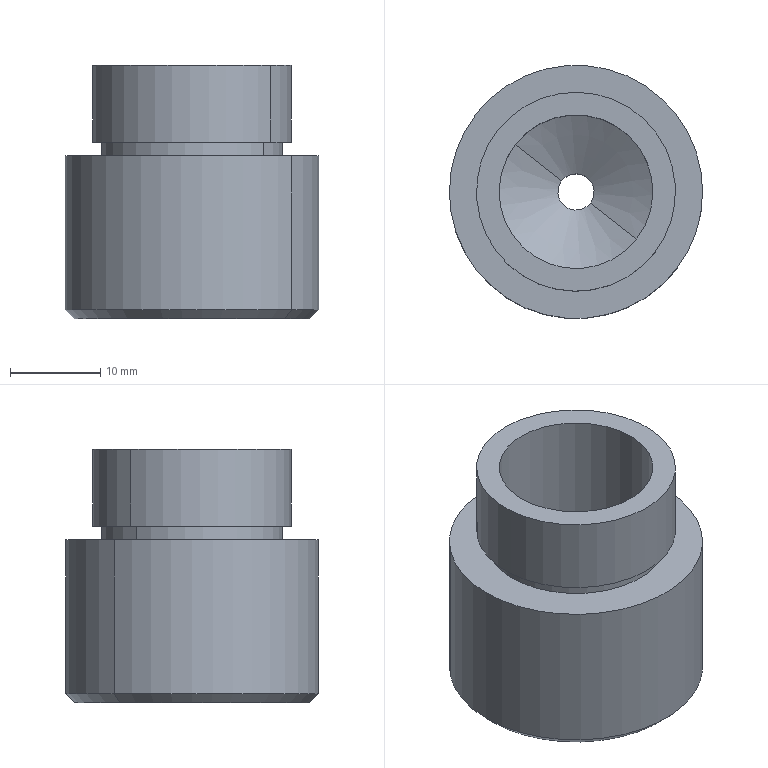Component | SolidWorks | 29-1 | 1 solid | 20 faces | box 28 x 28 x 28 mm | volume 11443 mm3 | cylinder 10 | cone 6 | plane 4 | commonest cylinder face diameters 28 x2 20 x2 22 x2 17 x2 4 x2
build123d program:
from build123d import *

# Parameters (mm, degrees)
CHAMFER1_SIZE = 1


with BuildPart() as part:
    # Sketch1 → Revolve1 (revolve)
    with BuildSketch(Plane.XY, mode=Mode.PRIVATE) as revolve1_sk:
        Polygon((14, 28), (4.5, 28), (2, 25.5), (2, 15.753), (8.5, 12), (8.5, 0), (11, 0), (11, 8.5), (10, 8.5), (10, 10), (14, 10), align=None)
    revolve(revolve1_sk.sketch.rotate(Axis((0, 0, 0), (0, 1, 0)), 90), axis=Axis((0, 0, 0), (0, 1, 0)))

    # Chamfer1
    chamfer1_edges = [part.edges().sort_by_distance(p)[0] for p in [
        (0, 28, 14),
    ]]
    chamfer(chamfer1_edges, length=CHAMFER1_SIZE)


solid = part.part

# Placed as in the assembly
solid = solid.moved(Location((-135.043, 380.991, 870.242), (-90, 0, 0)))
STEP:
#1=COLOUR_RGB('',0.7922,0.8196,0.9333);
#2=FILL_AREA_STYLE_COLOUR('',#1);
#3=FILL_AREA_STYLE('',(#2));
#4=SURFACE_STYLE_FILL_AREA(#3);
#5=SURFACE_SIDE_STYLE('',(#4));
#6=SURFACE_STYLE_USAGE(.BOTH.,#5);
#7=PRESENTATION_STYLE_ASSIGNMENT((#6));
#8=CARTESIAN_POINT('',(-5.72,15.315,33.159));
#9=VERTEX_POINT('',#8);
#10=CARTESIAN_POINT('',(-4.913,14.685,33.159));
#11=VERTEX_POINT('',#10);
#12=CARTESIAN_POINT('',(-5.317,15.,33.159));
#13=DIRECTION('',(-0.,-0.,-1.));
#14=DIRECTION('',(0.7882,-0.6155,0.));
#15=AXIS2_PLACEMENT_3D('',#12,#13,#14);
#16=CIRCLE('',#15,0.5118);
#17=EDGE_CURVE('',#9,#11,#16,.T.);
#18=ORIENTED_EDGE('',*,*,#17,.F.);
#19=CARTESIAN_POINT('',(-5.751,15.339,33.199));
#20=VERTEX_POINT('',#19);
#21=CARTESIAN_POINT('',(-5.751,15.339,33.199));
#22=DIRECTION('',(-0.5573,0.4352,0.7071));
#23=VECTOR('',#22,39.37);
#24=LINE('',#21,#23);
#25=EDGE_CURVE('',#9,#20,#24,.T.);
#26=ORIENTED_EDGE('',*,*,#25,.T.);
#27=CARTESIAN_POINT('',(-4.882,14.66,33.199));
#28=VERTEX_POINT('',#27);
#29=CARTESIAN_POINT('',(-5.317,15.,33.199));
#30=DIRECTION('',(0.,0.,1.));
#31=DIRECTION('',(0.7882,-0.6155,0.));
#32=AXIS2_PLACEMENT_3D('',#29,#30,#31);
#33=CIRCLE('',#32,0.5512);
#34=EDGE_CURVE('',#28,#20,#33,.T.);
#35=ORIENTED_EDGE('',*,*,#34,.F.);
#36=CARTESIAN_POINT('',(-4.882,14.66,33.199));
#37=DIRECTION('',(0.5573,-0.4352,0.7071));
#38=VECTOR('',#37,39.37);
#39=LINE('',#36,#38);
#40=EDGE_CURVE('',#11,#28,#39,.T.);
#41=ORIENTED_EDGE('',*,*,#40,.F.);
#42=EDGE_LOOP('',(#18,#26,#35,#41));
#43=FACE_OUTER_BOUND('',#42,.T.);
#44=CARTESIAN_POINT('',(-5.317,15.,33.199));
#45=DIRECTION('',(0.,0.,1.));
#46=DIRECTION('',(0.7882,-0.6155,0.));
#47=AXIS2_PLACEMENT_3D('',#44,#45,#46);
#48=CONICAL_SURFACE('',#47,0.5512,0.7854);
#49=ADVANCED_FACE('',(#43),#48,.T.);
#50=ORIENTED_EDGE('',*,*,#34,.T.);
#51=CARTESIAN_POINT('',(-5.751,15.339,33.868));
#52=VERTEX_POINT('',#51);
#53=CARTESIAN_POINT('',(-5.751,15.339,34.262));
#54=DIRECTION('',(0.,0.,1.));
#55=VECTOR('',#54,39.37);
#56=LINE('',#53,#55);
#57=EDGE_CURVE('',#20,#52,#56,.T.);
#58=ORIENTED_EDGE('',*,*,#57,.T.);
#59=CARTESIAN_POINT('',(-4.882,14.66,33.868));
#60=VERTEX_POINT('',#59);
#61=CARTESIAN_POINT('',(-5.317,15.,33.868));
#62=DIRECTION('',(0.,0.,1.));
#63=DIRECTION('',(0.7882,-0.6155,0.));
#64=AXIS2_PLACEMENT_3D('',#61,#62,#63);
#65=CIRCLE('',#64,0.5512);
#66=EDGE_CURVE('',#60,#52,#65,.T.);
#67=ORIENTED_EDGE('',*,*,#66,.F.);
#68=CARTESIAN_POINT('',(-4.882,14.66,34.262));
#69=DIRECTION('',(0.,0.,1.));
#70=VECTOR('',#69,39.37);
#71=LINE('',#68,#70);
#72=EDGE_CURVE('',#28,#60,#71,.T.);
#73=ORIENTED_EDGE('',*,*,#72,.F.);
#74=EDGE_LOOP('',(#50,#58,#67,#73));
#75=FACE_OUTER_BOUND('',#74,.T.);
#76=CARTESIAN_POINT('',(-5.317,15.,34.262));
#77=DIRECTION('',(0.,0.,1.));
#78=DIRECTION('',(0.7882,-0.6155,0.));
#79=AXIS2_PLACEMENT_3D('',#76,#77,#78);
#80=CYLINDRICAL_SURFACE('',#79,0.5512);
#81=ADVANCED_FACE('',(#75),#80,.T.);
#82=CARTESIAN_POINT('',(-5.006,14.757,33.868));
#83=VERTEX_POINT('',#82);
#84=CARTESIAN_POINT('',(-5.627,15.242,33.868));
#85=VERTEX_POINT('',#84);
#86=CARTESIAN_POINT('',(-5.317,15.,33.868));
#87=DIRECTION('',(0.,0.,1.));
#88=DIRECTION('',(0.7882,-0.6155,0.));
#89=AXIS2_PLACEMENT_3D('',#86,#87,#88);
#90=CIRCLE('',#89,0.3937);
#91=EDGE_CURVE('',#83,#85,#90,.T.);
#92=ORIENTED_EDGE('',*,*,#91,.T.);
#93=CARTESIAN_POINT('',(-5.627,15.242,33.927));
#94=VERTEX_POINT('',#93);
#95=CARTESIAN_POINT('',(-5.627,15.242,34.262));
#96=DIRECTION('',(0.,0.,1.));
#97=VECTOR('',#96,39.37);
#98=LINE('',#95,#97);
#99=EDGE_CURVE('',#85,#94,#98,.T.);
#100=ORIENTED_EDGE('',*,*,#99,.T.);
#101=CARTESIAN_POINT('',(-5.006,14.757,33.927));
#102=VERTEX_POINT('',#101);
#103=CARTESIAN_POINT('',(-5.317,15.,33.927));
#104=DIRECTION('',(0.,0.,1.));
#105=DIRECTION('',(0.7882,-0.6155,0.));
#106=AXIS2_PLACEMENT_3D('',#103,#104,#105);
#107=CIRCLE('',#106,0.3937);
#108=EDGE_CURVE('',#102,#94,#107,.T.);
#109=ORIENTED_EDGE('',*,*,#108,.F.);
#110=CARTESIAN_POINT('',(-5.006,14.757,34.262));
#111=DIRECTION('',(0.,0.,1.));
#112=VECTOR('',#111,39.37);
#113=LINE('',#110,#112);
#114=EDGE_CURVE('',#83,#102,#113,.T.);
#115=ORIENTED_EDGE('',*,*,#114,.F.);
#116=EDGE_LOOP('',(#92,#100,#109,#115));
#117=FACE_OUTER_BOUND('',#116,.T.);
#118=CARTESIAN_POINT('',(-5.317,15.,34.262));
#119=DIRECTION('',(0.,0.,1.));
#120=DIRECTION('',(0.7882,-0.6155,0.));
#121=AXIS2_PLACEMENT_3D('',#118,#119,#120);
#122=CYLINDRICAL_SURFACE('',#121,0.3937);
#123=ADVANCED_FACE('',(#117),#122,.T.);
#124=CARTESIAN_POINT('',(-4.975,14.733,33.927));
#125=VERTEX_POINT('',#124);
#126=CARTESIAN_POINT('',(-5.658,15.266,33.927));
#127=VERTEX_POINT('',#126);
#128=CARTESIAN_POINT('',(-5.317,15.,33.927));
#129=DIRECTION('',(0.,0.,1.));
#130=DIRECTION('',(0.7882,-0.6155,0.));
#131=AXIS2_PLACEMENT_3D('',#128,#129,#130);
#132=CIRCLE('',#131,0.4331);
#133=EDGE_CURVE('',#125,#127,#132,.T.);
#134=ORIENTED_EDGE('',*,*,#133,.T.);
#135=CARTESIAN_POINT('',(-5.658,15.266,34.262));
#136=VERTEX_POINT('',#135);
#137=CARTESIAN_POINT('',(-5.658,15.266,34.262));
#138=DIRECTION('',(0.,0.,1.));
#139=VECTOR('',#138,39.37);
#140=LINE('',#137,#139);
#141=EDGE_CURVE('',#127,#136,#140,.T.);
#142=ORIENTED_EDGE('',*,*,#141,.T.);
#143=CARTESIAN_POINT('',(-4.975,14.733,34.262));
#144=VERTEX_POINT('',#143);
#145=CARTESIAN_POINT('',(-5.317,15.,34.262));
#146=DIRECTION('',(0.,0.,1.));
#147=DIRECTION('',(0.7882,-0.6155,0.));
#148=AXIS2_PLACEMENT_3D('',#145,#146,#147);
#149=CIRCLE('',#148,0.4331);
#150=EDGE_CURVE('',#144,#136,#149,.T.);
#151=ORIENTED_EDGE('',*,*,#150,.F.);
#152=CARTESIAN_POINT('',(-4.975,14.733,34.262));
#153=DIRECTION('',(0.,0.,1.));
#154=VECTOR('',#153,39.37);
#155=LINE('',#152,#154);
#156=EDGE_CURVE('',#125,#144,#155,.T.);
#157=ORIENTED_EDGE('',*,*,#156,.F.);
#158=EDGE_LOOP('',(#134,#142,#151,#157));
#159=FACE_OUTER_BOUND('',#158,.T.);
#160=CARTESIAN_POINT('',(-5.317,15.,34.262));
#161=DIRECTION('',(0.,0.,1.));
#162=DIRECTION('',(0.7882,-0.6155,0.));
#163=AXIS2_PLACEMENT_3D('',#160,#161,#162);
#164=CYLINDRICAL_SURFACE('',#163,0.4331);
#165=ADVANCED_FACE('',(#159),#164,.T.);
#166=CARTESIAN_POINT('',(-5.58,15.206,33.789));
#167=VERTEX_POINT('',#166);
#168=CARTESIAN_POINT('',(-5.053,14.794,33.789));
#169=VERTEX_POINT('',#168);
#170=CARTESIAN_POINT('',(-5.317,15.,33.789));
#171=DIRECTION('',(0.,0.,1.));
#172=DIRECTION('',(0.7882,-0.6155,0.));
#173=AXIS2_PLACEMENT_3D('',#170,#171,#172);
#174=CIRCLE('',#173,0.3346);
#175=EDGE_CURVE('',#167,#169,#174,.T.);
#176=ORIENTED_EDGE('',*,*,#175,.F.);
#177=CARTESIAN_POINT('',(-5.58,15.206,34.262));
#178=VERTEX_POINT('',#177);
#179=CARTESIAN_POINT('',(-5.58,15.206,34.262));
#180=DIRECTION('',(0.,0.,1.));
#181=VECTOR('',#180,39.37);
#182=LINE('',#179,#181);
#183=EDGE_CURVE('',#167,#178,#182,.T.);
#184=ORIENTED_EDGE('',*,*,#183,.T.);
#185=CARTESIAN_POINT('',(-5.053,14.794,34.262));
#186=VERTEX_POINT('',#185);
#187=CARTESIAN_POINT('',(-5.317,15.,34.262));
#188=DIRECTION('',(0.,0.,1.));
#189=DIRECTION('',(0.7882,-0.6155,0.));
#190=AXIS2_PLACEMENT_3D('',#187,#188,#189);
#191=CIRCLE('',#190,0.3346);
#192=EDGE_CURVE('',#178,#186,#191,.T.);
#193=ORIENTED_EDGE('',*,*,#192,.T.);
#194=CARTESIAN_POINT('',(-5.053,14.794,34.262));
#195=DIRECTION('',(0.,0.,1.));
#196=VECTOR('',#195,39.37);
#197=LINE('',#194,#196);
#198=EDGE_CURVE('',#169,#186,#197,.T.);
#199=ORIENTED_EDGE('',*,*,#198,.F.);
#200=EDGE_LOOP('',(#176,#184,#193,#199));
#201=FACE_OUTER_BOUND('',#200,.T.);
#202=CARTESIAN_POINT('',(-5.317,15.,34.262));
#203=DIRECTION('',(0.,0.,1.));
#204=DIRECTION('',(0.7882,-0.6155,0.));
#205=AXIS2_PLACEMENT_3D('',#202,#203,#204);
#206=CYLINDRICAL_SURFACE('',#205,0.3346);
#207=ADVANCED_FACE('',(#201),#206,.F.);
#208=CARTESIAN_POINT('',(-5.379,15.048,33.641));
#209=VERTEX_POINT('',#208);
#210=CARTESIAN_POINT('',(-5.255,14.951,33.641));
#211=VERTEX_POINT('',#210);
#212=CARTESIAN_POINT('',(-5.317,15.,33.641));
#213=DIRECTION('',(0.,0.,1.));
#214=DIRECTION('',(0.7882,-0.6155,0.));
#215=AXIS2_PLACEMENT_3D('',#212,#213,#214);
#216=CIRCLE('',#215,0.07874);
#217=EDGE_CURVE('',#209,#211,#216,.T.);
#218=ORIENTED_EDGE('',*,*,#217,.F.);
#219=CARTESIAN_POINT('',(-5.58,15.206,33.789));
#220=DIRECTION('',(-0.6826,0.533,0.5));
#221=VECTOR('',#220,39.37);
#222=LINE('',#219,#221);
#223=EDGE_CURVE('',#209,#167,#222,.T.);
#224=ORIENTED_EDGE('',*,*,#223,.T.);
#225=ORIENTED_EDGE('',*,*,#175,.T.);
#226=CARTESIAN_POINT('',(-5.053,14.794,33.789));
#227=DIRECTION('',(0.6826,-0.533,0.5));
#228=VECTOR('',#227,39.37);
#229=LINE('',#226,#228);
#230=EDGE_CURVE('',#211,#169,#229,.T.);
#231=ORIENTED_EDGE('',*,*,#230,.F.);
#232=EDGE_LOOP('',(#218,#224,#225,#231));
#233=FACE_OUTER_BOUND('',#232,.T.);
#234=CARTESIAN_POINT('',(-5.317,15.,33.789));
#235=DIRECTION('',(0.,0.,1.));
#236=DIRECTION('',(0.7882,-0.6155,0.));
#237=AXIS2_PLACEMENT_3D('',#234,#235,#236);
#238=CONICAL_SURFACE('',#237,0.3346,1.047);
#239=ADVANCED_FACE('',(#233),#238,.F.);
#240=CARTESIAN_POINT('',(-5.379,15.048,33.258));
#241=VERTEX_POINT('',#240);
#242=CARTESIAN_POINT('',(-5.255,14.951,33.258));
#243=VERTEX_POINT('',#242);
#244=CARTESIAN_POINT('',(-5.317,15.,33.258));
#245=DIRECTION('',(0.,0.,1.));
#246=DIRECTION('',(0.7882,-0.6155,0.));
#247=AXIS2_PLACEMENT_3D('',#244,#245,#246);
#248=CIRCLE('',#247,0.07874);
#249=EDGE_CURVE('',#241,#243,#248,.T.);
#250=ORIENTED_EDGE('',*,*,#249,.F.);
#251=CARTESIAN_POINT('',(-5.379,15.048,34.262));
#252=DIRECTION('',(0.,0.,1.));
#253=VECTOR('',#252,39.37);
#254=LINE('',#251,#253);
#255=EDGE_CURVE('',#241,#209,#254,.T.);
#256=ORIENTED_EDGE('',*,*,#255,.T.);
#257=ORIENTED_EDGE('',*,*,#217,.T.);
#258=CARTESIAN_POINT('',(-5.255,14.951,34.262));
#259=DIRECTION('',(0.,0.,1.));
#260=VECTOR('',#259,39.37);
#261=LINE('',#258,#260);
#262=EDGE_CURVE('',#243,#211,#261,.T.);
#263=ORIENTED_EDGE('',*,*,#262,.F.);
#264=EDGE_LOOP('',(#250,#256,#257,#263));
#265=FACE_OUTER_BOUND('',#264,.T.);
#266=CARTESIAN_POINT('',(-5.317,15.,34.262));
#267=DIRECTION('',(0.,0.,1.));
#268=DIRECTION('',(0.7882,-0.6155,0.));
#269=AXIS2_PLACEMENT_3D('',#266,#267,#268);
#270=CYLINDRICAL_SURFACE('',#269,0.07874);
#271=ADVANCED_FACE('',(#265),#270,.F.);
#272=ORIENTED_EDGE('',*,*,#249,.T.);
#273=CARTESIAN_POINT('',(-5.177,14.891,33.159));
#274=VERTEX_POINT('',#273);
#275=CARTESIAN_POINT('',(-5.255,14.951,33.258));
#276=DIRECTION('',(0.5573,-0.4352,-0.7071));
#277=VECTOR('',#276,39.37);
#278=LINE('',#275,#277);
#279=EDGE_CURVE('',#243,#274,#278,.T.);
#280=ORIENTED_EDGE('',*,*,#279,.T.);
#281=CARTESIAN_POINT('',(-5.456,15.109,33.159));
#282=VERTEX_POINT('',#281);
#283=CARTESIAN_POINT('',(-5.317,15.,33.159));
#284=DIRECTION('',(0.,0.,1.));
#285=DIRECTION('',(0.7882,-0.6155,0.));
#286=AXIS2_PLACEMENT_3D('',#283,#284,#285);
#287=CIRCLE('',#286,0.1772);
#288=EDGE_CURVE('',#282,#274,#287,.T.);
#289=ORIENTED_EDGE('',*,*,#288,.F.);
#290=CARTESIAN_POINT('',(-5.379,15.048,33.258));
#291=DIRECTION('',(-0.5573,0.4352,-0.7071));
#292=VECTOR('',#291,39.37);
#293=LINE('',#290,#292);
#294=EDGE_CURVE('',#241,#282,#293,.T.);
#295=ORIENTED_EDGE('',*,*,#294,.F.);
#296=EDGE_LOOP('',(#272,#280,#289,#295));
#297=FACE_OUTER_BOUND('',#296,.T.);
#298=CARTESIAN_POINT('',(-5.317,15.,33.258));
#299=DIRECTION('',(-0.,-0.,-1.));
#300=DIRECTION('',(-0.7882,0.6155,0.));
#301=AXIS2_PLACEMENT_3D('',#298,#299,#300);
#302=CONICAL_SURFACE('',#301,0.07874,0.7854);
#303=ADVANCED_FACE('',(#297),#302,.F.);
#304=ORIENTED_EDGE('',*,*,#279,.F.);
#305=CARTESIAN_POINT('',(-5.317,15.,33.258));
#306=DIRECTION('',(0.,0.,1.));
#307=DIRECTION('',(0.7882,-0.6155,0.));
#308=AXIS2_PLACEMENT_3D('',#305,#306,#307);
#309=CIRCLE('',#308,0.07874);
#310=EDGE_CURVE('',#243,#241,#309,.T.);
#311=ORIENTED_EDGE('',*,*,#310,.T.);
#312=ORIENTED_EDGE('',*,*,#294,.T.);
#313=CARTESIAN_POINT('',(-5.317,15.,33.159));
#314=DIRECTION('',(0.,0.,1.));
#315=DIRECTION('',(0.7882,-0.6155,0.));
#316=AXIS2_PLACEMENT_3D('',#313,#314,#315);
#317=CIRCLE('',#316,0.1772);
#318=EDGE_CURVE('',#274,#282,#317,.T.);
#319=ORIENTED_EDGE('',*,*,#318,.F.);
#320=EDGE_LOOP('',(#304,#311,#312,#319));
#321=FACE_OUTER_BOUND('',#320,.T.);
#322=CARTESIAN_POINT('',(-5.317,15.,33.258));
#323=DIRECTION('',(-0.,-0.,-1.));
#324=DIRECTION('',(-0.7882,0.6155,0.));
#325=AXIS2_PLACEMENT_3D('',#322,#323,#324);
#326=CONICAL_SURFACE('',#325,0.07874,0.7854);
#327=ADVANCED_FACE('',(#321),#326,.F.);
#328=ORIENTED_EDGE('',*,*,#255,.F.);
#329=ORIENTED_EDGE('',*,*,#310,.F.);
#330=ORIENTED_EDGE('',*,*,#262,.T.);
#331=CARTESIAN_POINT('',(-5.317,15.,33.641));
#332=DIRECTION('',(0.,0.,1.));
#333=DIRECTION('',(0.7882,-0.6155,0.));
#334=AXIS2_PLACEMENT_3D('',#331,#332,#333);
#335=CIRCLE('',#334,0.07874);
#336=EDGE_CURVE('',#211,#209,#335,.T.);
#337=ORIENTED_EDGE('',*,*,#336,.T.);
#338=EDGE_LOOP('',(#328,#329,#330,#337));
#339=FACE_OUTER_BOUND('',#338,.T.);
#340=CARTESIAN_POINT('',(-5.317,15.,34.262));
#341=DIRECTION('',(0.,0.,1.));
#342=DIRECTION('',(0.7882,-0.6155,0.));
#343=AXIS2_PLACEMENT_3D('',#340,#341,#342);
#344=CYLINDRICAL_SURFACE('',#343,0.07874);
#345=ADVANCED_FACE('',(#339),#344,.F.);
#346=ORIENTED_EDGE('',*,*,#223,.F.);
#347=ORIENTED_EDGE('',*,*,#336,.F.);
#348=ORIENTED_EDGE('',*,*,#230,.T.);
#349=CARTESIAN_POINT('',(-5.317,15.,33.789));
#350=DIRECTION('',(0.,0.,1.));
#351=DIRECTION('',(0.7882,-0.6155,0.));
#352=AXIS2_PLACEMENT_3D('',#349,#350,#351);
#353=CIRCLE('',#352,0.3346);
#354=EDGE_CURVE('',#169,#167,#353,.T.);
#355=ORIENTED_EDGE('',*,*,#354,.T.);
#356=EDGE_LOOP('',(#346,#347,#348,#355));
#357=FACE_OUTER_BOUND('',#356,.T.);
#358=CARTESIAN_POINT('',(-5.317,15.,33.789));
#359=DIRECTION('',(0.,0.,1.));
#360=DIRECTION('',(0.7882,-0.6155,0.));
#361=AXIS2_PLACEMENT_3D('',#358,#359,#360);
#362=CONICAL_SURFACE('',#361,0.3346,1.047);
#363=ADVANCED_FACE('',(#357),#362,.F.);
#364=ORIENTED_EDGE('',*,*,#183,.F.);
#365=ORIENTED_EDGE('',*,*,#354,.F.);
#366=ORIENTED_EDGE('',*,*,#198,.T.);
#367=CARTESIAN_POINT('',(-5.317,15.,34.262));
#368=DIRECTION('',(0.,0.,1.));
#369=DIRECTION('',(0.7882,-0.6155,0.));
#370=AXIS2_PLACEMENT_3D('',#367,#368,#369);
#371=CIRCLE('',#370,0.3346);
#372=EDGE_CURVE('',#186,#178,#371,.T.);
#373=ORIENTED_EDGE('',*,*,#372,.T.);
#374=EDGE_LOOP('',(#364,#365,#366,#373));
#375=FACE_OUTER_BOUND('',#374,.T.);
#376=CARTESIAN_POINT('',(-5.317,15.,34.262));
#377=DIRECTION('',(0.,0.,1.));
#378=DIRECTION('',(0.7882,-0.6155,0.));
#379=AXIS2_PLACEMENT_3D('',#376,#377,#378);
#380=CYLINDRICAL_SURFACE('',#379,0.3346);
#381=ADVANCED_FACE('',(#375),#380,.F.);
#382=ORIENTED_EDGE('',*,*,#372,.F.);
#383=ORIENTED_EDGE('',*,*,#192,.F.);
#384=EDGE_LOOP('',(#382,#383));
#385=FACE_BOUND('',#384,.T.);
#386=ORIENTED_EDGE('',*,*,#150,.T.);
#387=CARTESIAN_POINT('',(-5.317,15.,34.262));
#388=DIRECTION('',(0.,0.,1.));
#389=DIRECTION('',(0.7882,-0.6155,0.));
#390=AXIS2_PLACEMENT_3D('',#387,#388,#389);
#391=CIRCLE('',#390,0.4331);
#392=EDGE_CURVE('',#136,#144,#391,.T.);
#393=ORIENTED_EDGE('',*,*,#392,.T.);
#394=EDGE_LOOP('',(#386,#393));
#395=FACE_OUTER_BOUND('',#394,.T.);
#396=CARTESIAN_POINT('',(-5.317,15.,34.262));
#397=DIRECTION('',(-0.,-0.,-1.));
#398=DIRECTION('',(-0.7882,0.6155,0.));
#399=AXIS2_PLACEMENT_3D('',#396,#397,#398);
#400=PLANE('',#399);
#401=ADVANCED_FACE('',(#385,#395),#400,.F.);
#402=ORIENTED_EDGE('',*,*,#141,.F.);
#403=CARTESIAN_POINT('',(-5.317,15.,33.927));
#404=DIRECTION('',(0.,0.,1.));
#405=DIRECTION('',(0.7882,-0.6155,0.));
#406=AXIS2_PLACEMENT_3D('',#403,#404,#405);
#407=CIRCLE('',#406,0.4331);
#408=EDGE_CURVE('',#127,#125,#407,.T.);
#409=ORIENTED_EDGE('',*,*,#408,.T.);
#410=ORIENTED_EDGE('',*,*,#156,.T.);
#411=ORIENTED_EDGE('',*,*,#392,.F.);
#412=EDGE_LOOP('',(#402,#409,#410,#411));
#413=FACE_OUTER_BOUND('',#412,.T.);
#414=CARTESIAN_POINT('',(-5.317,15.,34.262));
#415=DIRECTION('',(0.,0.,1.));
#416=DIRECTION('',(0.7882,-0.6155,0.));
#417=AXIS2_PLACEMENT_3D('',#414,#415,#416);
#418=CYLINDRICAL_SURFACE('',#417,0.4331);
#419=ADVANCED_FACE('',(#413),#418,.T.);
#420=ORIENTED_EDGE('',*,*,#133,.F.);
#421=ORIENTED_EDGE('',*,*,#408,.F.);
#422=EDGE_LOOP('',(#420,#421));
#423=FACE_OUTER_BOUND('',#422,.T.);
#424=ORIENTED_EDGE('',*,*,#108,.T.);
#425=CARTESIAN_POINT('',(-5.317,15.,33.927));
#426=DIRECTION('',(0.,0.,1.));
#427=DIRECTION('',(0.7882,-0.6155,0.));
#428=AXIS2_PLACEMENT_3D('',#425,#426,#427);
#429=CIRCLE('',#428,0.3937);
#430=EDGE_CURVE('',#94,#102,#429,.T.);
#431=ORIENTED_EDGE('',*,*,#430,.T.);
#432=EDGE_LOOP('',(#424,#431));
#433=FACE_BOUND('',#432,.T.);
#434=CARTESIAN_POINT('',(-5.317,15.,33.927));
#435=DIRECTION('',(0.,0.,1.));
#436=DIRECTION('',(0.7882,-0.6155,-0.));
#437=AXIS2_PLACEMENT_3D('',#434,#435,#436);
#438=PLANE('',#437);
#439=ADVANCED_FACE('',(#423,#433),#438,.F.);
#440=ORIENTED_EDGE('',*,*,#99,.F.);
#441=CARTESIAN_POINT('',(-5.317,15.,33.868));
#442=DIRECTION('',(0.,0.,1.));
#443=DIRECTION('',(0.7882,-0.6155,0.));
#444=AXIS2_PLACEMENT_3D('',#441,#442,#443);
#445=CIRCLE('',#444,0.3937);
#446=EDGE_CURVE('',#85,#83,#445,.T.);
#447=ORIENTED_EDGE('',*,*,#446,.T.);
#448=ORIENTED_EDGE('',*,*,#114,.T.);
#449=ORIENTED_EDGE('',*,*,#430,.F.);
#450=EDGE_LOOP('',(#440,#447,#448,#449));
#451=FACE_OUTER_BOUND('',#450,.T.);
#452=CARTESIAN_POINT('',(-5.317,15.,34.262));
#453=DIRECTION('',(0.,0.,1.));
#454=DIRECTION('',(0.7882,-0.6155,0.));
#455=AXIS2_PLACEMENT_3D('',#452,#453,#454);
#456=CYLINDRICAL_SURFACE('',#455,0.3937);
#457=ADVANCED_FACE('',(#451),#456,.T.);
#458=ORIENTED_EDGE('',*,*,#91,.F.);
#459=ORIENTED_EDGE('',*,*,#446,.F.);
#460=EDGE_LOOP('',(#458,#459));
#461=FACE_BOUND('',#460,.T.);
#462=ORIENTED_EDGE('',*,*,#66,.T.);
#463=CARTESIAN_POINT('',(-5.317,15.,33.868));
#464=DIRECTION('',(0.,0.,1.));
#465=DIRECTION('',(0.7882,-0.6155,0.));
#466=AXIS2_PLACEMENT_3D('',#463,#464,#465);
#467=CIRCLE('',#466,0.5512);
#468=EDGE_CURVE('',#52,#60,#467,.T.);
#469=ORIENTED_EDGE('',*,*,#468,.T.);
#470=EDGE_LOOP('',(#462,#469));
#471=FACE_OUTER_BOUND('',#470,.T.);
#472=CARTESIAN_POINT('',(-5.317,15.,33.868));
#473=DIRECTION('',(-0.,-0.,-1.));
#474=DIRECTION('',(-0.7882,0.6155,0.));
#475=AXIS2_PLACEMENT_3D('',#472,#473,#474);
#476=PLANE('',#475);
#477=ADVANCED_FACE('',(#461,#471),#476,.F.);
#478=ORIENTED_EDGE('',*,*,#57,.F.);
#479=CARTESIAN_POINT('',(-5.317,15.,33.199));
#480=DIRECTION('',(0.,0.,1.));
#481=DIRECTION('',(0.7882,-0.6155,0.));
#482=AXIS2_PLACEMENT_3D('',#479,#480,#481);
#483=CIRCLE('',#482,0.5512);
#484=EDGE_CURVE('',#20,#28,#483,.T.);
#485=ORIENTED_EDGE('',*,*,#484,.T.);
#486=ORIENTED_EDGE('',*,*,#72,.T.);
#487=ORIENTED_EDGE('',*,*,#468,.F.);
#488=EDGE_LOOP('',(#478,#485,#486,#487));
#489=FACE_OUTER_BOUND('',#488,.T.);
#490=CARTESIAN_POINT('',(-5.317,15.,34.262));
#491=DIRECTION('',(0.,0.,1.));
#492=DIRECTION('',(0.7882,-0.6155,0.));
#493=AXIS2_PLACEMENT_3D('',#490,#491,#492);
#494=CYLINDRICAL_SURFACE('',#493,0.5512);
#495=ADVANCED_FACE('',(#489),#494,.T.);
#496=CARTESIAN_POINT('',(-5.317,15.,33.159));
#497=DIRECTION('',(-0.,-0.,-1.));
#498=DIRECTION('',(0.7882,-0.6155,0.));
#499=AXIS2_PLACEMENT_3D('',#496,#497,#498);
#500=CIRCLE('',#499,0.5118);
#501=EDGE_CURVE('',#11,#9,#500,.T.);
#502=ORIENTED_EDGE('',*,*,#501,.T.);
#503=ORIENTED_EDGE('',*,*,#17,.T.);
#504=EDGE_LOOP('',(#502,#503));
#505=FACE_OUTER_BOUND('',#504,.T.);
#506=ORIENTED_EDGE('',*,*,#288,.T.);
#507=ORIENTED_EDGE('',*,*,#318,.T.);
#508=EDGE_LOOP('',(#506,#507));
#509=FACE_BOUND('',#508,.T.);
#510=CARTESIAN_POINT('',(-5.317,15.,33.159));
#511=DIRECTION('',(0.,0.,1.));
#512=DIRECTION('',(0.7882,-0.6155,-0.));
#513=AXIS2_PLACEMENT_3D('',#510,#511,#512);
#514=PLANE('',#513);
#515=ADVANCED_FACE('',(#505,#509),#514,.F.);
#516=ORIENTED_EDGE('',*,*,#25,.F.);
#517=ORIENTED_EDGE('',*,*,#501,.F.);
#518=ORIENTED_EDGE('',*,*,#40,.T.);
#519=ORIENTED_EDGE('',*,*,#484,.F.);
#520=EDGE_LOOP('',(#516,#517,#518,#519));
#521=FACE_OUTER_BOUND('',#520,.T.);
#522=CARTESIAN_POINT('',(-5.317,15.,33.199));
#523=DIRECTION('',(0.,0.,1.));
#524=DIRECTION('',(0.7882,-0.6155,0.));
#525=AXIS2_PLACEMENT_3D('',#522,#523,#524);
#526=CONICAL_SURFACE('',#525,0.5512,0.7854);
#527=ADVANCED_FACE('',(#521),#526,.T.);
#528=CLOSED_SHELL('',(#49,#81,#123,#165,#207,#239,#271,#303,#327,#345,#363,#381,#401,#419,#439,#457,#477,#495,#515,#527));
#529=MANIFOLD_SOLID_BREP('',#528);
#530=STYLED_ITEM('',(#7),#529);
#531=(LENGTH_UNIT()NAMED_UNIT(*)SI_UNIT($,.METRE.));
#532=LENGTH_MEASURE_WITH_UNIT(LENGTH_MEASURE(0.0254),#531);
#533=DIMENSIONAL_EXPONENTS(1.,0.,0.,0.,0.,0.,0.);
#534=(CONVERSION_BASED_UNIT('',#532)LENGTH_UNIT()NAMED_UNIT(#533));
#535=UNCERTAINTY_MEASURE_WITH_UNIT(LENGTH_MEASURE(0.00001),#534,'','');
#536=(NAMED_UNIT(*)PLANE_ANGLE_UNIT()SI_UNIT($,.RADIAN.));
#537=(NAMED_UNIT(*)SI_UNIT($,.STERADIAN.)SOLID_ANGLE_UNIT());
#538=(GEOMETRIC_REPRESENTATION_CONTEXT(3)GLOBAL_UNCERTAINTY_ASSIGNED_CONTEXT((#535))GLOBAL_UNIT_ASSIGNED_CONTEXT((#534,#536,#537))REPRESENTATION_CONTEXT('',''));
#539=MECHANICAL_DESIGN_GEOMETRIC_PRESENTATION_REPRESENTATION('',(#530),#538);
#540=CARTESIAN_POINT('',(0.,0.,0.));
#541=DIRECTION('',(0.,0.,1.));
#542=DIRECTION('',(1.,0.,0.));
#543=AXIS2_PLACEMENT_3D('',#540,#541,#542);
#544=(LENGTH_UNIT()NAMED_UNIT(*)SI_UNIT($,.METRE.));
#545=LENGTH_MEASURE_WITH_UNIT(LENGTH_MEASURE(0.0254),#544);
#546=DIMENSIONAL_EXPONENTS(1.,0.,0.,0.,0.,0.,0.);
#547=(CONVERSION_BASED_UNIT('',#545)LENGTH_UNIT()NAMED_UNIT(#546));
#548=UNCERTAINTY_MEASURE_WITH_UNIT(LENGTH_MEASURE(0.00001),#547,'','');
#549=(NAMED_UNIT(*)PLANE_ANGLE_UNIT()SI_UNIT($,.RADIAN.));
#550=(NAMED_UNIT(*)SI_UNIT($,.STERADIAN.)SOLID_ANGLE_UNIT());
#551=(GEOMETRIC_REPRESENTATION_CONTEXT(3)GLOBAL_UNCERTAINTY_ASSIGNED_CONTEXT((#548))GLOBAL_UNIT_ASSIGNED_CONTEXT((#547,#549,#550))REPRESENTATION_CONTEXT('',''));
#552=ADVANCED_BREP_SHAPE_REPRESENTATION('',(#529,#543),#551);
#553=PRESENTATION_LAYER_ASSIGNMENT('','',(#530));